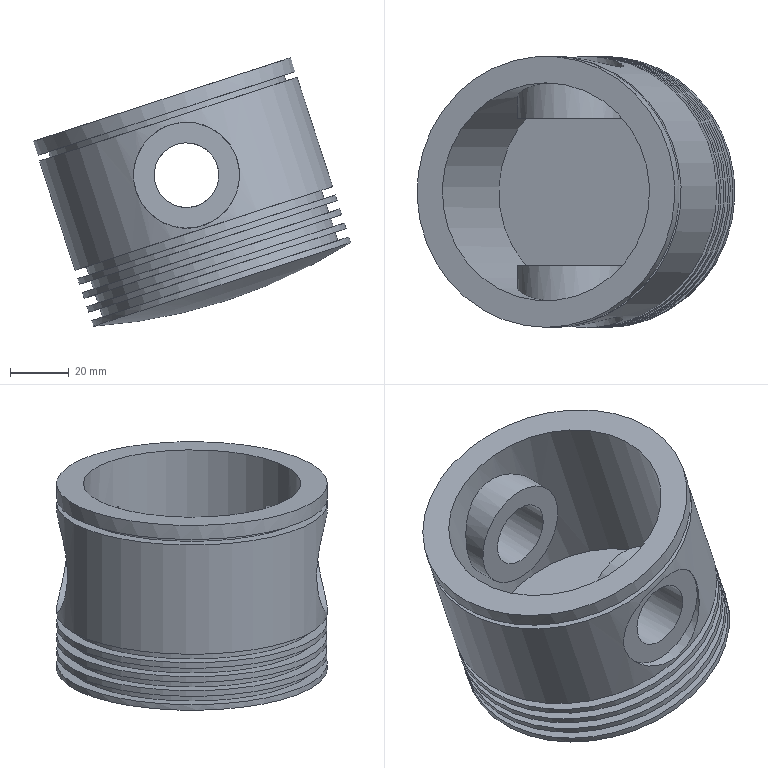Component | NX | RADIAL_ENGINE_4 | 1 solid | 35 faces | volume 178484 mm3 | cylinder 18 | plane 16 | sphere 1 | commonest cylinder face diameters 92 x6 84 x5 36 x4 22 x2 74 x1